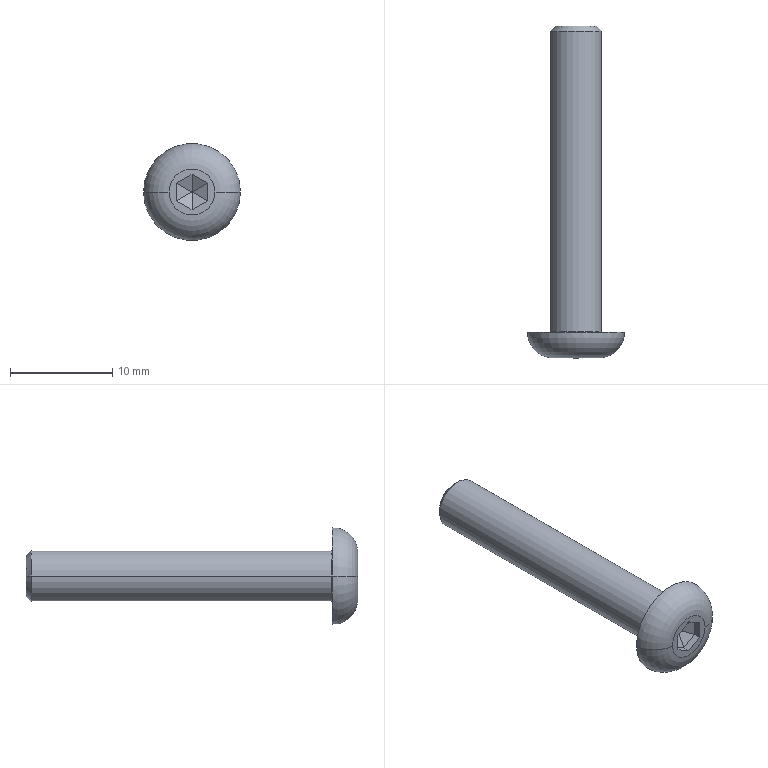Component | SolidWorks | SocketHeadCapScrewM5x30-1 | 1 solid | 24 faces | volume 721 mm3 | plane 16 | torus 4 | cone 2 | cylinder 2 | commonest cylinder face diameters 5 x2 | material Plain Carbon Steel